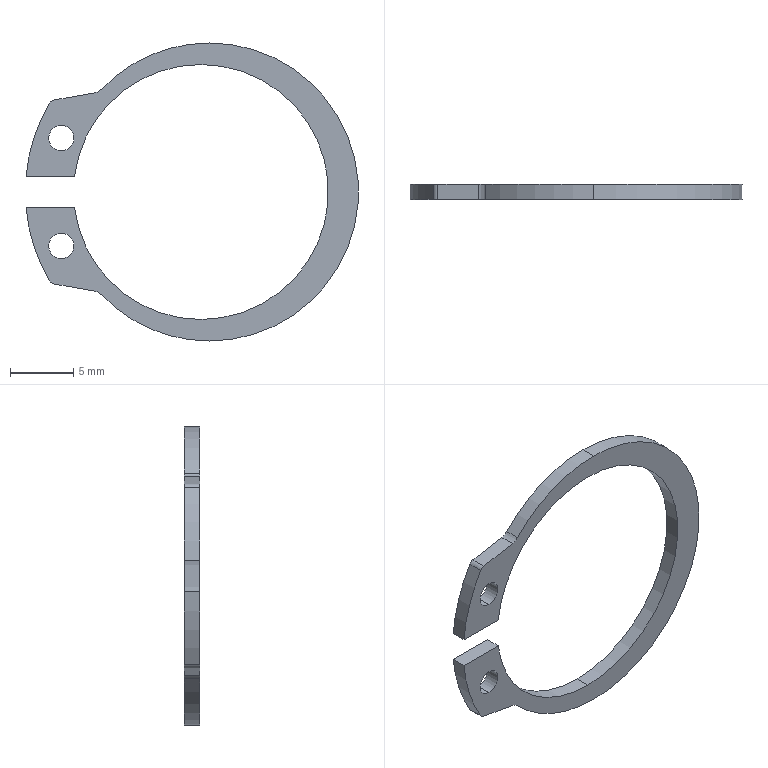Component | SolidWorks | JL001-05-03-1_GB_T894-2017[RetainingRingForShaftA-type(d0_10)21]-2 | 1 solid | 22 faces | box 26.21 x 1.2 x 23.5 mm | volume 174 mm3 | cylinder 16 | plane 6 | commonest cylinder face diameters 2 x6 23.5 x3 20.1 x3 1 x2 27.7 x2
build123d program:
from build123d import *

# Parameters (mm, degrees)
BASE_EXTRUDE_DEPTH      = 0.6
BASE_EXTRUDE_DEPTH_BACK = 0.6
SKETCH1_R               = 1


with BuildPart() as part:
    # Sketch1 → Base-Extrude (new, two sides: drawn at the far end of the back side and taken through both)
    with BuildSketch(Plane.XY.offset(-BASE_EXTRUDE_DEPTH_BACK)):
        with BuildLine():
            Line((-1.25, -10.642), (-1.25, -14.463))
            ThreePointArc((-1.25, -14.463), (-4.233, -13.857), (-7.011, -12.615))
            ThreePointArc((-7.011, -12.615), (-7.168, -12.469), (-7.25, -12.27))
            Line((-7.25, -12.27), (-7.818, -9.05))
            ThreePointArc((-7.818, -9.05), (-7.921, -8.752), (-8.112, -8.5))
            ThreePointArc((-8.112, -8.5), (0, 11.75), (8.112, -8.5))
            ThreePointArc((8.112, -8.5), (7.921, -8.752), (7.818, -9.05))
            Line((7.818, -9.05), (7.25, -12.27))
            ThreePointArc((7.25, -12.27), (7.168, -12.469), (7.011, -12.615))
            ThreePointArc((7.011, -12.615), (4.233, -13.857), (1.25, -14.463))
            Line((1.25, -14.463), (1.25, -10.642))
            ThreePointArc((1.25, -10.642), (0, 9.38), (-1.25, -10.642))
        make_face()
        with Locations((-4.25, -11.678)):
            Circle(SKETCH1_R, mode=Mode.SUBTRACT)
        with Locations(Location((4.25, -11.678, 0), (0, 0, 180))):
            Circle(SKETCH1_R, mode=Mode.SUBTRACT)
    extrude(amount=BASE_EXTRUDE_DEPTH + BASE_EXTRUDE_DEPTH_BACK)


solid = part.part

# Placed as in the assembly
solid = solid.moved(Location((0.67, 302.948, 105), (90, 0, -90)))